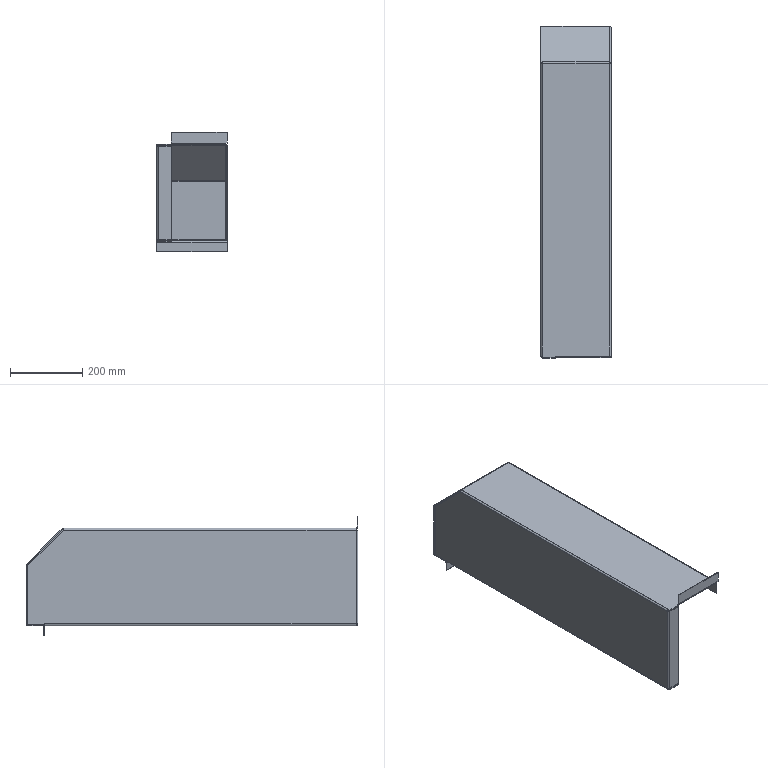Component | NX | SIDE_COLUMN_FRONT_LEFT | 1 solid | 93 faces | volume 1115598 mm3 | plane 70 | cylinder 23 | commonest cylinder face diameters 6 x12 10 x11